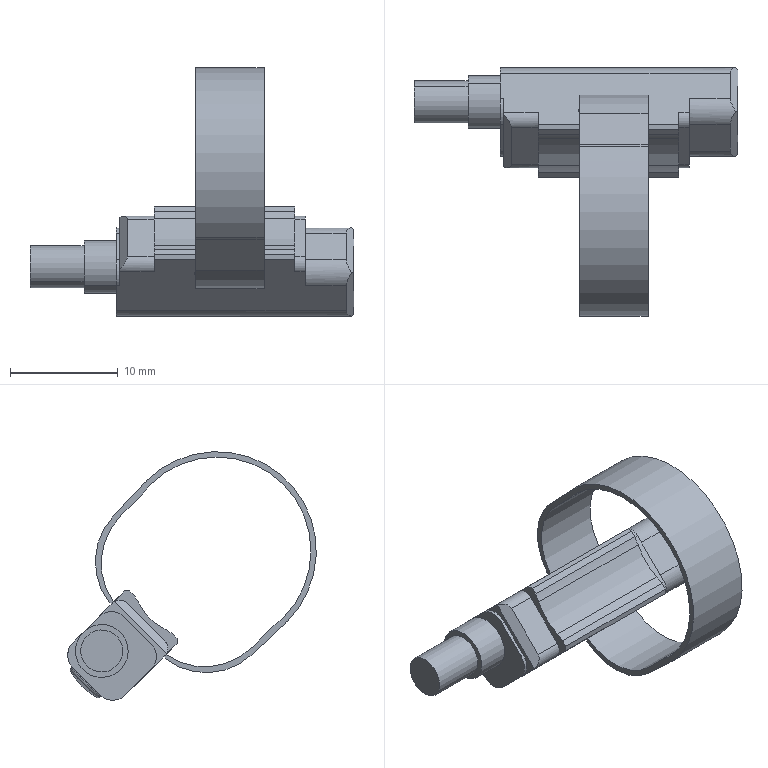Component | SolidWorks | 17268PB16x60SU(58)+(CS1-M-2)-1_17268CS1-M-S16-1 | 1 solid | 72 faces | box 30 x 23.03 x 23.03 mm | volume 1454 mm3 | plane 39 | cylinder 29 | sphere 2 | torus 2 | commonest cylinder face diameters 3.4 x6 17.4 x5 12.4 x4 2 x4 18.4 x3 3.8 x2 3.9 x2 4.9 x2
build123d program:
from build123d import *

# Parameters (mm, degrees)
BOSS_EXTRUDE1_DEPTH               = 3.175
BOSS_EXTRUDE1_DEPTH_BACK          = 3.175
BOSS_EXTRUDE2_DEPTH               = 18.5
CUT_EXTRUDE1_DEPTH                = 4.5
CUT_EXTRUDE2_DEPTH                = 5.5
CUT_EXTRUDE3_DEPTH                = 18.5
BOSS_EXTRUDE3_DEPTH               = 3.5
CUT_EXTRUDE4_DEPTH                = 3.25
CUT_EXTRUDE4_DEPTH_BACK           = 3.25
SKETCH7_W                         = 7.3
SKETCH7_H                         = 0.3
SKETCH8_R                         = 2.45
BOSS_EXTRUDE4_DEPTH               = 25
SKETCH9_R                         = 1.95
BOSS_EXTRUDE5_DEPTH               = 30
BOSS_EXTRUDE6_DEPTH               = 3.2
CUT_EXTRUDE5_DEPTH                = 5
CUT_EXTRUDE5_DEPTH_BACK           = 5
CUT_EXTRUDE6_DEPTH                = 5
CUT_EXTRUDE6_DEPTH_BACK           = 5
CUT_EXTRUDE7_DEPTH                = 10
CUT_EXTRUDE7_DEPTH_BACK           = 10
THREAD_FIT_RELIEF_BAND_DEPTH      = 28.206
THREAD_FIT_RELIEF_BAND_DEPTH_BACK = 28.206
SKETCH1_R                         = 8.7


with BuildPart() as part:
    # Sketch1_2 → Boss-Extrude1 (new, two sides: drawn at the far end of the back side and taken through both)
    with BuildSketch(Plane(origin=(11.5, 0, 0), x_dir=(0, 0, -1), z_dir=(1, 0, 0)).offset(-BOSS_EXTRUDE1_DEPTH_BACK)):
        with BuildLine():
            Line((9.196, 0.2661), (9.074, 4.479))
            ThreePointArc((9.074, 4.479), (7.197, 8.747), (2.877, 10.5))
            Line((2.877, 10.5), (-2.877, 10.5))
            ThreePointArc((-2.877, 10.5), (-7.197, 8.747), (-9.074, 4.479))
            Line((-9.074, 4.479), (-9.196, 0.2661))
            ThreePointArc((-9.196, 0.2661), (0, -9.2), (9.196, 0.2661))
        make_face()
        with BuildLine():
            Line((8.6, 0), (8.6, 4))
            ThreePointArc((8.6, 4), (6.784, 8.384), (2.4, 10.2))
            Line((2.4, 10.2), (-2.4, 10.2))
            ThreePointArc((-2.4, 10.2), (-6.784, 8.384), (-8.6, 4))
            Line((-8.6, 4), (-8.6, 0))
            ThreePointArc((-8.6, 0), (0, -8.6), (8.6, 0))
        make_face(mode=Mode.SUBTRACT)
    extrude(amount=BOSS_EXTRUDE1_DEPTH + BOSS_EXTRUDE1_DEPTH_BACK)

    # Sketch2 → Boss-Extrude2 (add)
    with BuildSketch(Plane(origin=(0, 0, 0), x_dir=(0, 0, -1), z_dir=(1, 0, 0))):
        with BuildLine():
            Line((-3.45, 15.4), (-3.45, 8.687))
            Line((-3.45, 8.687), (-3.096, 8.333))
            Line((-3.096, 8.333), (-2.5, 8.333))
            Line((-2.5, 8.333), (-2.5, 8))
            Line((-2.5, 8), (2.5, 8))
            Line((2.5, 8), (2.5, 8.333))
            Line((2.5, 8.333), (3.096, 8.333))
            Line((3.096, 8.333), (3.45, 8.687))
            Line((3.45, 8.687), (3.45, 15.4))
            ThreePointArc((3.45, 15.4), (2.952, 16.602), (1.75, 17.1))
            Line((1.75, 17.1), (-1.75, 17.1))
            ThreePointArc((-1.75, 17.1), (-2.952, 16.602), (-3.45, 15.4))
        make_face()
    extrude(amount=BOSS_EXTRUDE2_DEPTH)

    # Sketch3 → Cut-Extrude1 (cut)
    with BuildSketch(Plane(origin=(0, 0, 0), x_dir=(0, 0, -1), z_dir=(1, 0, 0))):
        with BuildLine():
            Line((-3.45, 12.1), (-3.45, 8.687))
            Line((-3.45, 8.687), (-3.096, 8.333))
            Line((-3.096, 8.333), (-2.5, 8.333))
            Line((-2.5, 8.333), (-2.5, 8))
            Line((-2.5, 8), (2.5, 8))
            Line((2.5, 8), (2.5, 8.333))
            Line((2.5, 8.333), (3.096, 8.333))
            Line((3.096, 8.333), (3.45, 8.687))
            Line((3.45, 8.687), (3.45, 12.1))
            ThreePointArc((3.45, 12.1), (2.952, 10.898), (1.75, 10.4))
            Line((1.75, 10.4), (-1.75, 10.4))
            ThreePointArc((-1.75, 10.4), (-2.952, 10.898), (-3.45, 12.1))
        make_face()
    extrude(amount=CUT_EXTRUDE1_DEPTH, mode=Mode.SUBTRACT)

    # Sketch4 → Cut-Extrude2 (cut)
    with BuildSketch(Plane(origin=(0, 0, 0), x_dir=(0, 0, -1), z_dir=(1, 0, 0))):
        with BuildLine():
            Line((-3.45, 8.687), (-3.096, 8.333))
            Line((-3.096, 8.333), (-2.5, 8.333))
            Line((-2.5, 8.333), (-2.5, 8))
            Line((-2.5, 8), (2.5, 8))
            Line((2.5, 8), (2.5, 8.333))
            Line((2.5, 8.333), (3.096, 8.333))
            Line((3.096, 8.333), (3.45, 8.687))
            Line((3.45, 8.687), (3.45, 10.3))
            ThreePointArc((3.45, 10.3), (3.157, 9.593), (2.45, 9.3))
            Line((2.45, 9.3), (-2.45, 9.3))
            ThreePointArc((-2.45, 9.3), (-3.157, 9.593), (-3.45, 10.3))
            Line((-3.45, 10.3), (-3.45, 8.687))
        make_face()
    extrude(amount=CUT_EXTRUDE2_DEPTH, mode=Mode.SUBTRACT)

    # Sketch5 → Cut-Extrude3 (cut)
    with BuildSketch(Plane(origin=(0, 0, 0), x_dir=(0, 0, -1), z_dir=(1, 0, 0))):
        with BuildLine():
            Line((-2.5, 8.333), (-2.5, 7.6))
            Line((-2.5, 7.6), (2.5, 7.6))
            Line((2.5, 7.6), (2.5, 8.333))
            Line((2.5, 8.333), (2.18, 8.333))
            ThreePointArc((2.18, 8.333), (0, 8.833), (-2.18, 8.333))
            Line((-2.18, 8.333), (-2.5, 8.333))
        make_face()
    extrude(amount=CUT_EXTRUDE3_DEPTH, mode=Mode.SUBTRACT)

    # Sketch6 → Boss-Extrude3 (add)
    with BuildSketch(Plane(origin=(18.5, 0, 0), x_dir=(0, 0, -1), z_dir=(1, 0, 0))):
        with BuildLine():
            Line((-1.75, 10.4), (1.75, 10.4))
            ThreePointArc((1.75, 10.4), (2.952, 10.898), (3.45, 12.1))
            Line((3.45, 12.1), (3.45, 15.4))
            ThreePointArc((3.45, 15.4), (2.952, 16.602), (1.75, 17.1))
            Line((1.75, 17.1), (-1.75, 17.1))
            ThreePointArc((-1.75, 17.1), (-2.952, 16.602), (-3.45, 15.4))
            Line((-3.45, 15.4), (-3.45, 12.1))
            ThreePointArc((-3.45, 12.1), (-2.952, 10.898), (-1.75, 10.4))
        make_face()
    extrude(amount=BOSS_EXTRUDE3_DEPTH)

    # Sketch7 → Cut-Extrude4 (cut, two sides: drawn at the far end of the back side and taken through both)
    with BuildSketch(Plane(origin=(11.5, 0, 0), x_dir=(0, 0, -1), z_dir=(1, 0, 0)).offset(-CUT_EXTRUDE4_DEPTH_BACK)):
        with Locations((0, 10.55)):
            Rectangle(SKETCH7_W, SKETCH7_H)
    extrude(amount=CUT_EXTRUDE4_DEPTH + CUT_EXTRUDE4_DEPTH_BACK, mode=Mode.SUBTRACT)

    # Sketch8 → Boss-Extrude4 (add)
    with BuildSketch(Plane(origin=(0, 0, 0), x_dir=(0, 0, -1), z_dir=(1, 0, 0))):
        with Locations((1, 14.1)):
            Circle(SKETCH8_R)
    extrude(amount=BOSS_EXTRUDE4_DEPTH)

    # Sketch9 → Boss-Extrude5 (add)
    with BuildSketch(Plane(origin=(0, 0, 0), x_dir=(0, 0, -1), z_dir=(1, 0, 0))):
        with Locations((1, 14.1)):
            Circle(SKETCH9_R)
    extrude(amount=BOSS_EXTRUDE5_DEPTH)

    # Sketch10 → Boss-Extrude6 (add)
    with BuildSketch(Plane(origin=(18.5, 0, 0), x_dir=(0, 0, -1), z_dir=(1, 0, 0))):
        with BuildLine():
            Line((-3.45, 12.1), (-3.45, 10.3))
            ThreePointArc((-3.45, 10.3), (-3.157, 9.593), (-2.45, 9.3))
            Line((-2.45, 9.3), (2.45, 9.3))
            ThreePointArc((2.45, 9.3), (3.157, 9.593), (3.45, 10.3))
            Line((3.45, 10.3), (3.45, 12.1))
            ThreePointArc((3.45, 12.1), (2.952, 10.898), (1.75, 10.4))
            Line((1.75, 10.4), (-1.75, 10.4))
            ThreePointArc((-1.75, 10.4), (-2.952, 10.898), (-3.45, 12.1))
        make_face()
    extrude(amount=BOSS_EXTRUDE6_DEPTH)

    # Sketch11 → Cut-Extrude5 (cut, two sides: drawn at the far end of the back side and taken through both)
    with BuildSketch(Plane.XY.offset(-CUT_EXTRUDE5_DEPTH_BACK)):
        Polygon((20.993, 9.3), (20.993, 8.3), (22.7, 8.3), (22.7, 10.007), (21.7, 10.007), align=None)
    extrude(amount=CUT_EXTRUDE5_DEPTH + CUT_EXTRUDE5_DEPTH_BACK, mode=Mode.SUBTRACT)

    # Sketch12 → Cut-Extrude6 (cut, two sides: drawn at the far end of the back side and taken through both)
    with BuildSketch(Plane.XY.offset(-CUT_EXTRUDE6_DEPTH_BACK)):
        Polygon((-1, 18.1), (-1, 9.4), (0.7071, 9.4), (0.7071, 10.4), (0, 11.107), (0, 16.393), (0.7071, 17.1), (0.7071, 18.1), align=None)
    extrude(amount=CUT_EXTRUDE6_DEPTH + CUT_EXTRUDE6_DEPTH_BACK, mode=Mode.SUBTRACT)

    # Sketch13 → Cut-Extrude7 (cut, two sides: drawn at the far end of the back side and taken through both)
    with BuildSketch(Plane(origin=(0, 17.1, 0), x_dir=(1, 0, 0), z_dir=(0, 1, 0)).offset(-CUT_EXTRUDE7_DEPTH_BACK)):
        Polygon((-1, -4.45), (0.7071, -4.45), (0.7071, -3.45), (0, -2.743), (0, 2.743), (0.7071, 3.45), (0.7071, 4.45), (-1, 4.45), align=None)
    extrude(amount=CUT_EXTRUDE7_DEPTH + CUT_EXTRUDE7_DEPTH_BACK, mode=Mode.SUBTRACT)

    # Sketch14 → Revolve1 (revolve)
    with BuildSketch(Plane(origin=(7.1, 0, 0), x_dir=(0, 0, -1), z_dir=(1, 0, 0)), mode=Mode.PRIVATE) as revolve1_sk:
        with BuildLine():
            Line((0, 17.1), (-1.9, 17.1))
            Line((-1.9, 17.1), (-1.9, 17.215))
            ThreePointArc((-1.9, 17.215), (-1.85, 17.366), (-1.72, 17.456))
            ThreePointArc((-1.72, 17.456), (-0.8685, 17.639), (0, 17.7))
            Line((0, 17.7), (0, 17.1))
        make_face()
    revolve(revolve1_sk.sketch.rotate(Axis((7.1, 17.7, 0), (0, -1, 0)), 180), axis=Axis((7.1, 17.7, 0), (0, -1, 0)))

    # Sketch1 → Thread fit relief band (cut, two sides: drawn at the far end of the back side and taken through both)
    with BuildSketch(Plane(origin=(18.5, 0, 0), x_dir=(0, 0, -1), z_dir=(1, 0, 0)).offset(-THREAD_FIT_RELIEF_BAND_DEPTH_BACK)):
        Circle(SKETCH1_R)
    extrude(amount=THREAD_FIT_RELIEF_BAND_DEPTH + THREAD_FIT_RELIEF_BAND_DEPTH_BACK, mode=Mode.SUBTRACT)


solid = part.part

# Placed as in the assembly
solid = solid.moved(Location((-91.8, -27.579, 21.5), (135, 0, -180)))